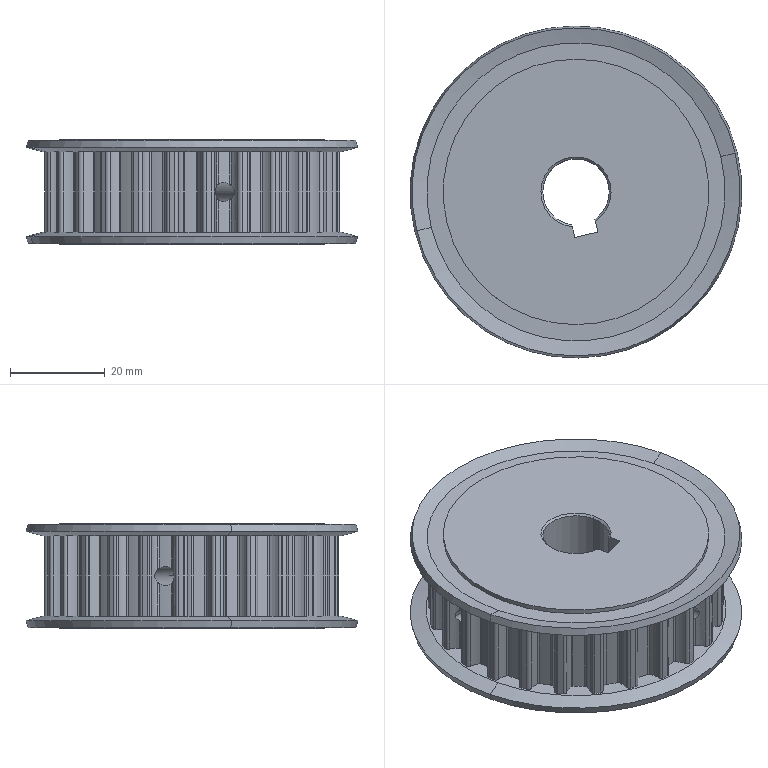Component | SolidWorks | CarrierZDG0406-A03-B02-X1-1 | 1 solid | 267 faces | volume 58914 mm3 | cylinder 240 | cone 18 | plane 9 | commonest cylinder face diameters 1.5 x61 0.8 x61 10.6 x53 56.63 x27 62.29 x25 56 x4 4.134 x4 14 x3 | material 45#